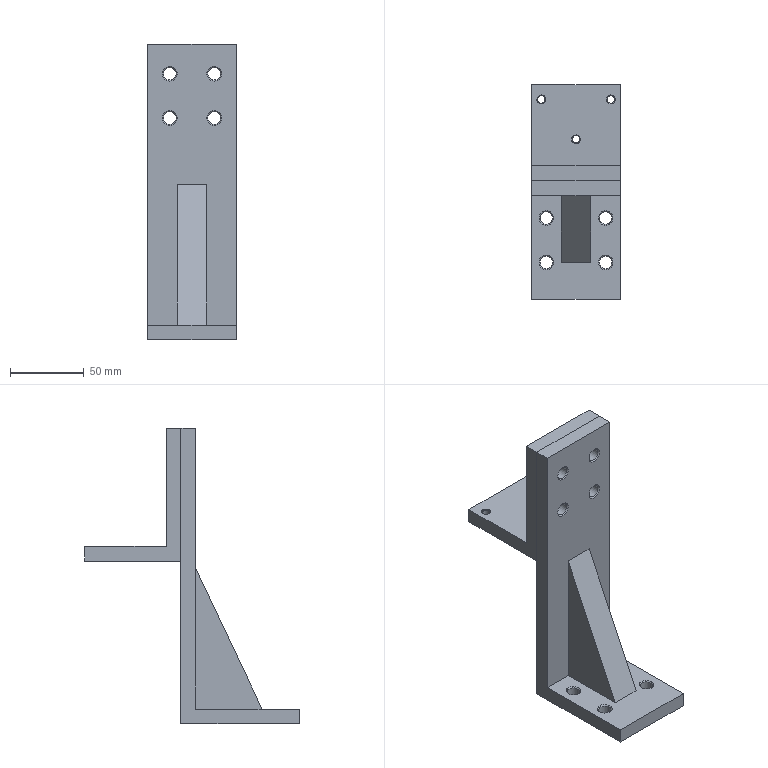Component | NX | Root-owned geometry | 3 solids | 86 faces | volume 279917 mm3 | cone 34 | cylinder 27 | plane 25 | commonest cylinder face diameters 8.5 x12 6.6 x4 11 x4 6 x4 5 x3